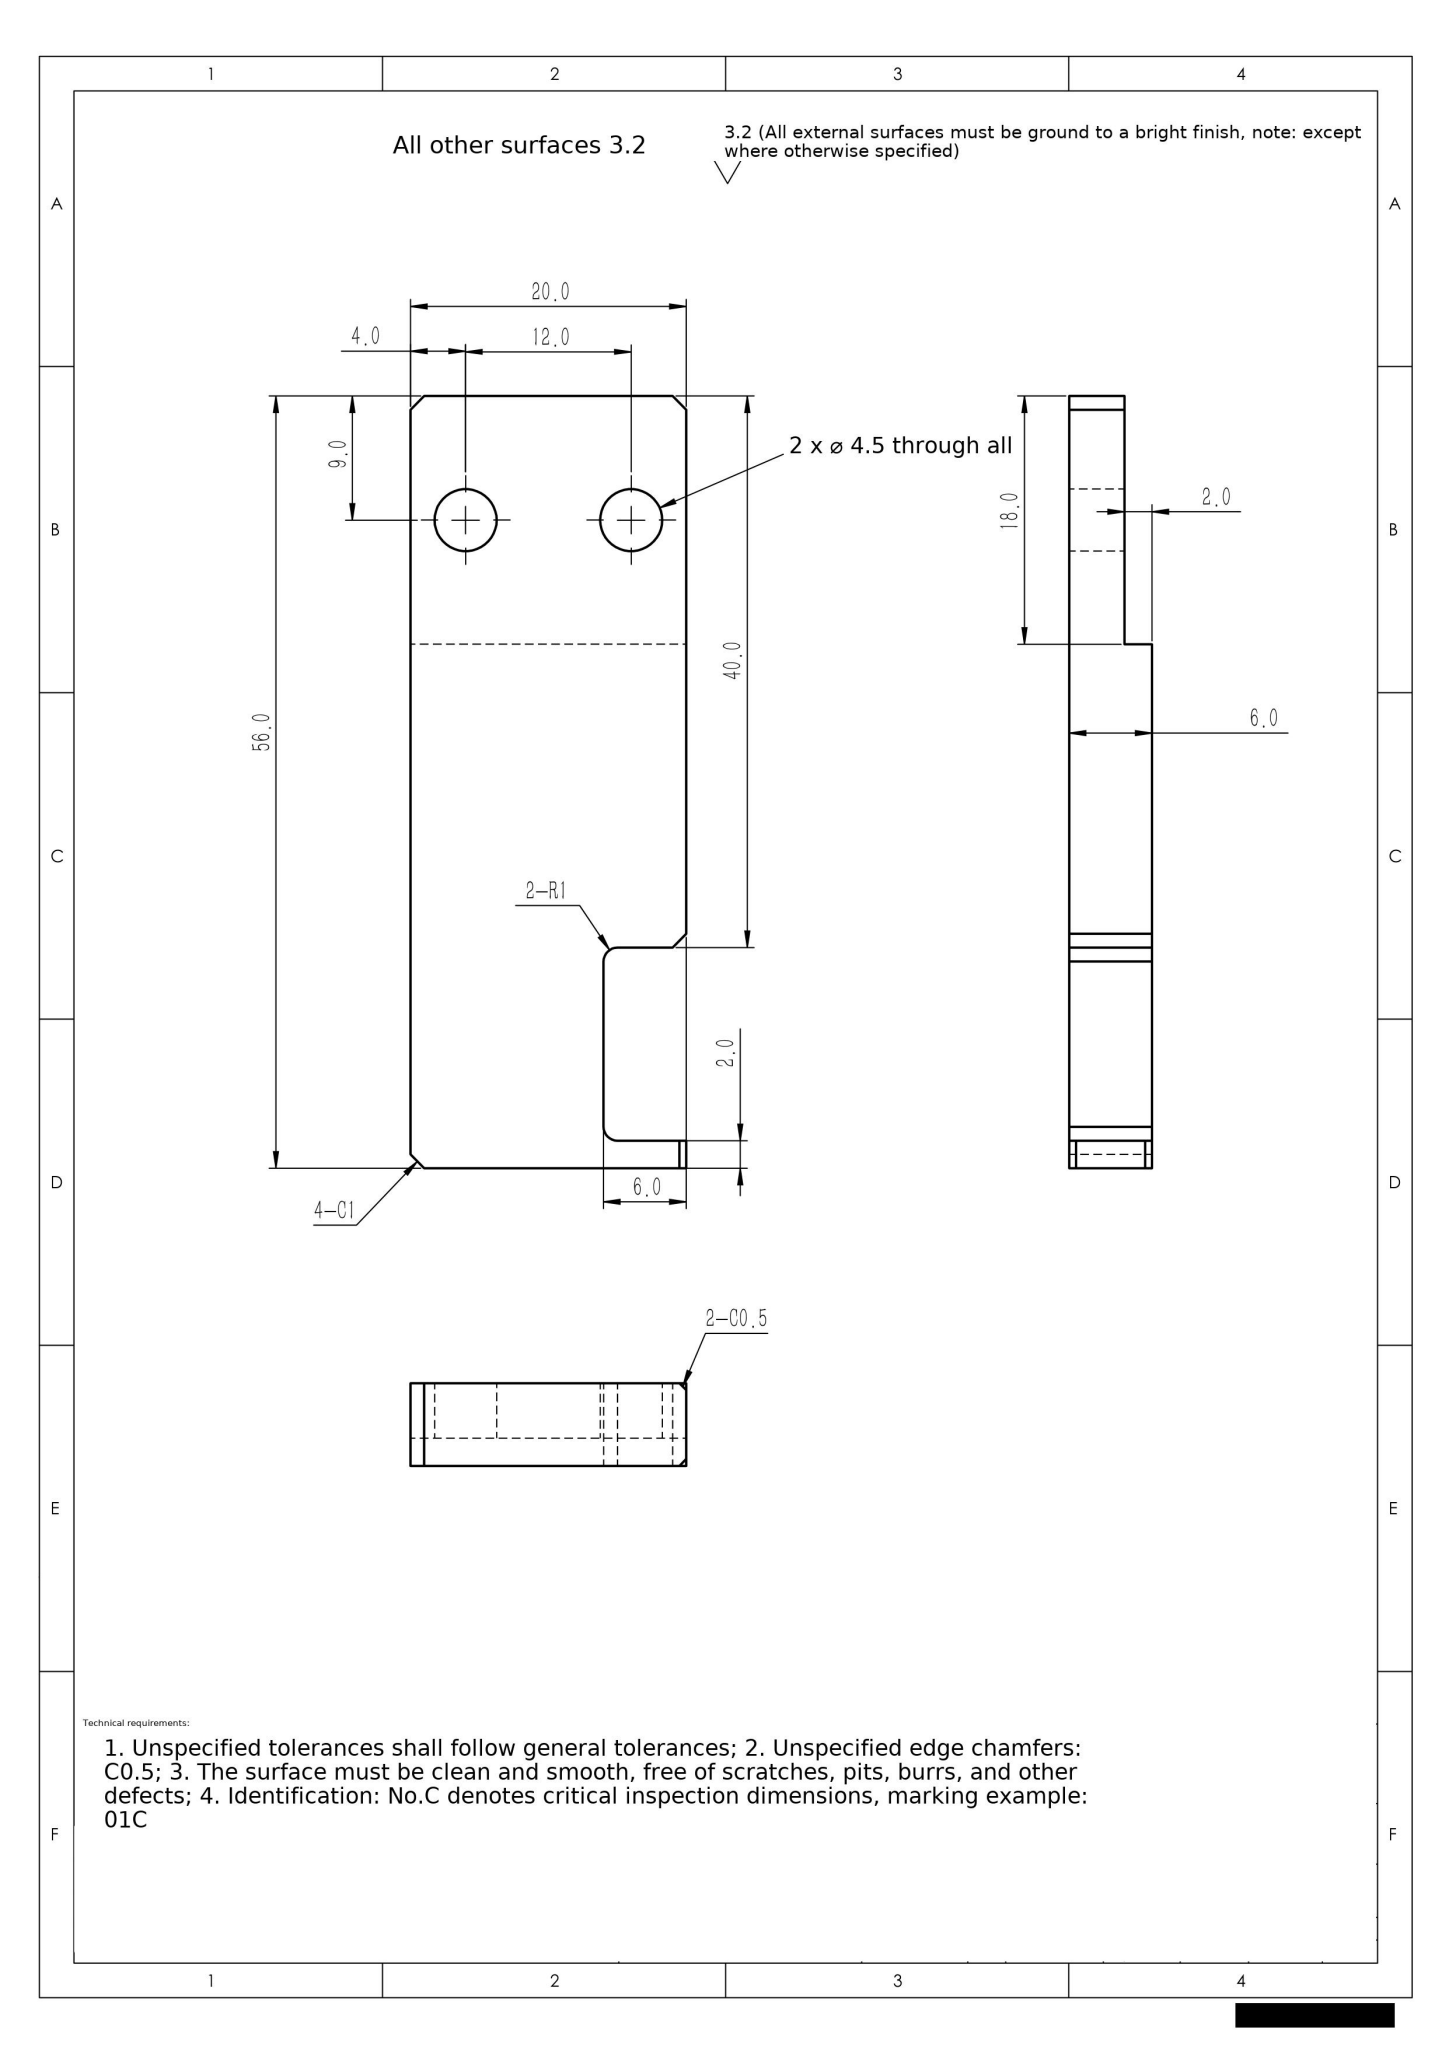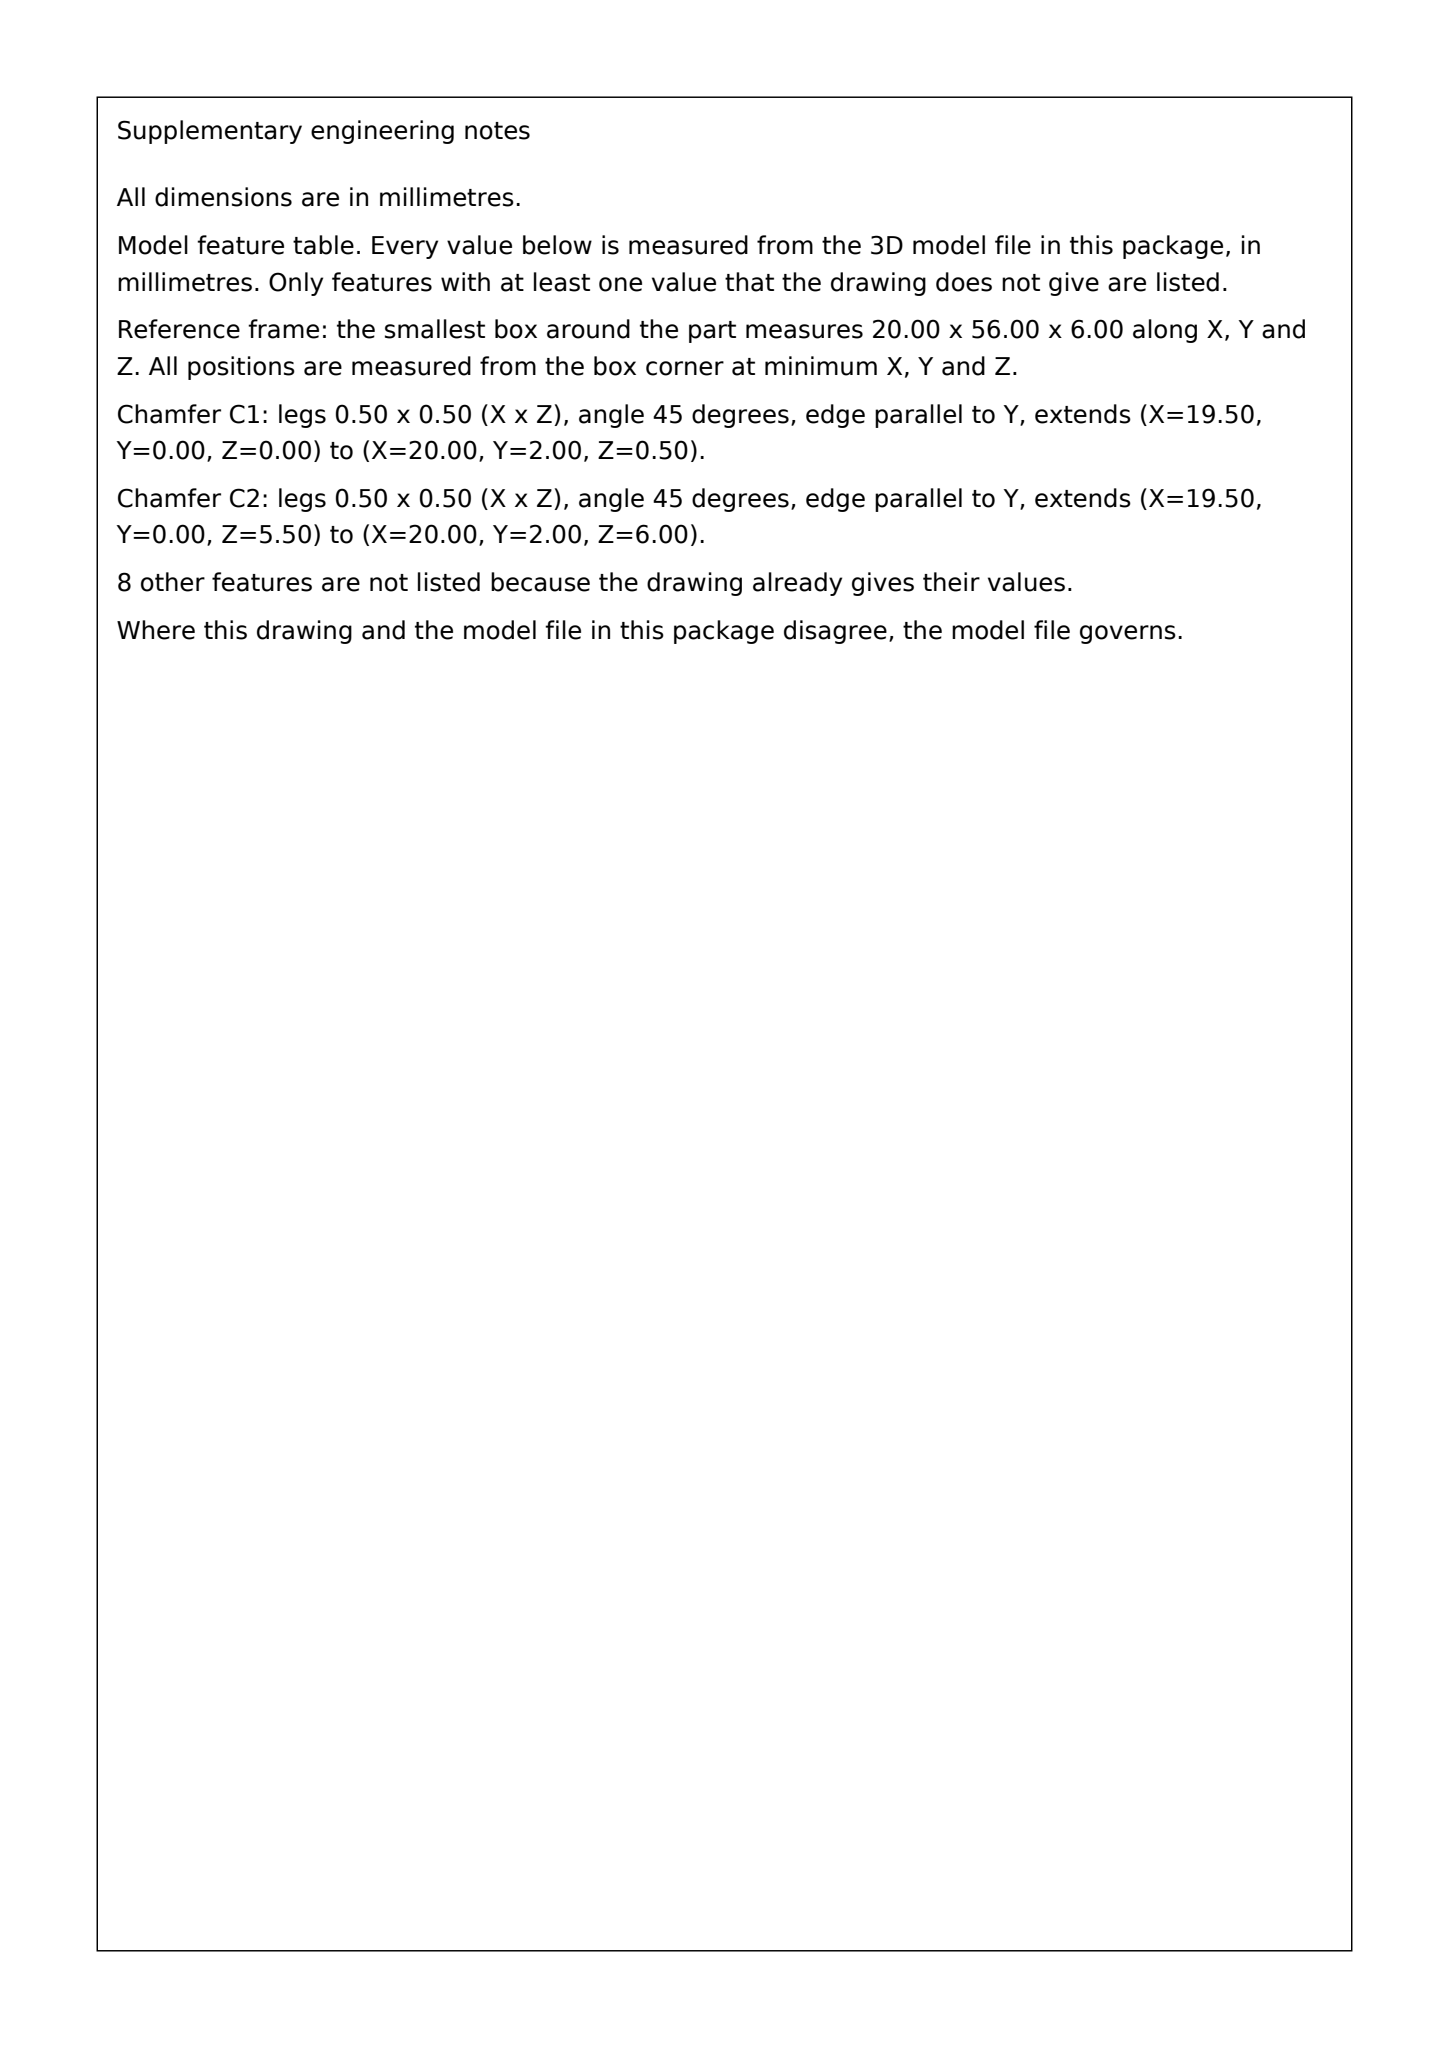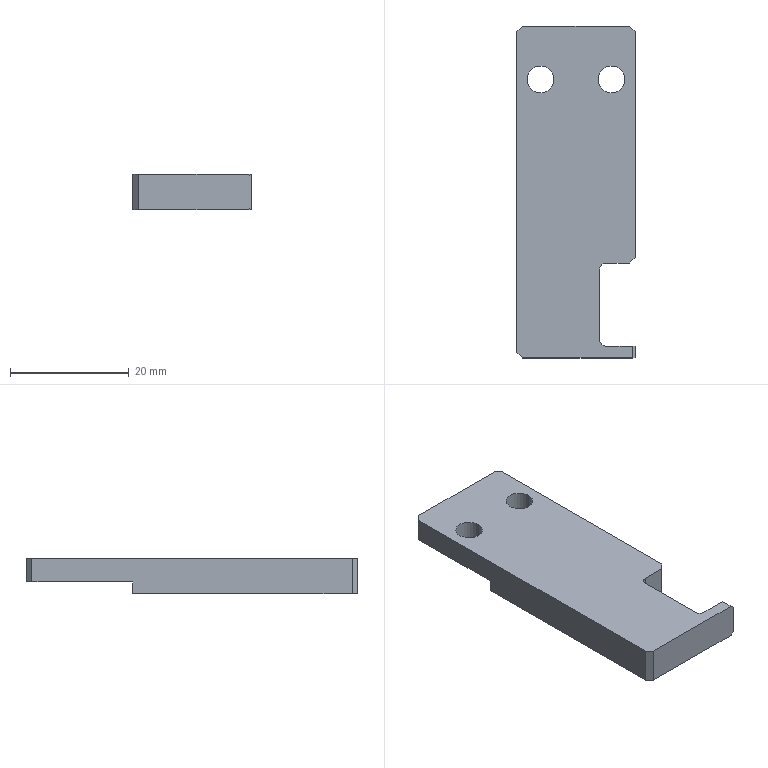Part | SolidWorks | mm | 1 solid | 24 faces | box 20 x 56 x 6 mm | volume 5361 mm3 | plane 18 | cylinder 6 | commonest cylinder face diameters 4.5 x4 2 x2
build123d program:
from build123d import *

# Parameters (mm, degrees)
SKETCH1_W                  = 20
SKETCH1_H                  = 56
BOSS_EXTRUDE1_DEPTH        = 3
F_4_5_4_5_DIAMETER_HOLE2_D = 4.5
SKETCH9_W                  = 6
SKETCH9_H                  = 14
CUT_EXTRUDE1_DEPTH         = 60.766
SKETCH10_W                 = 20
SKETCH10_H                 = 18
CUT_EXTRUDE2_DEPTH         = 2
CHAMFER1_SIZE              = 1
FILLET1_R                  = 1
CHAMFER2_SIZE              = 0.5


with BuildPart() as part:
    # Sketch1 → Boss-Extrude1 (new, symmetric)
    with BuildSketch(Plane.XY):
        with Locations((-10, 28)):
            Rectangle(SKETCH1_W, SKETCH1_H)
    extrude(amount=BOSS_EXTRUDE1_DEPTH, both=True)

    # 4.5 _4.5_ Diameter Hole2 (through all)
    with Locations(Plane(origin=(0, 0, -3), x_dir=(-1, 0, 0), z_dir=(0, 0, -1))):
        with Locations((4, 47), (16, 47)):
            Hole(F_4_5_4_5_DIAMETER_HOLE2_D / 2)

    # Sketch9 → Cut-Extrude1 (cut, through all)
    with BuildSketch(Plane.XY.offset(3)):
        with Locations((-3, 9)):
            Rectangle(SKETCH9_W, SKETCH9_H)
    extrude(amount=-CUT_EXTRUDE1_DEPTH, mode=Mode.SUBTRACT)

    # Sketch10 → Cut-Extrude2 (cut)
    with BuildSketch(Plane(origin=(0, 0, -3), x_dir=(-1, 0, 0), z_dir=(0, 0, -1))):
        with Locations((10, 47)):
            Rectangle(SKETCH10_W, SKETCH10_H)
    extrude(amount=-CUT_EXTRUDE2_DEPTH, mode=Mode.SUBTRACT)

    # Chamfer1
    chamfer1_edges = [part.edges().sort_by_distance(p)[0] for p in [
        (0, 16, 0),
        (-20, 0, 0),
        (-20, 56, 1),
        (0, 56, 1),
    ]]
    chamfer(chamfer1_edges, length=CHAMFER1_SIZE)

    # Fillet1
    fillet1_edges = [part.edges().sort_by_distance(p)[0] for p in [
        (-6, 2, 0),
        (-6, 16, 0),
    ]]
    fillet(fillet1_edges, radius=FILLET1_R)

    # Chamfer2
    chamfer2_edges = [part.edges().sort_by_distance(p)[0] for p in [
        (0, 1, 3),
        (0, 1, -3),
    ]]
    chamfer(chamfer2_edges, length=CHAMFER2_SIZE)


solid = part.part
STEP:
#1=CARTESIAN_POINT('',(-1.75,47.,3.));
#2=VERTEX_POINT('',#1);
#3=CARTESIAN_POINT('',(-6.25,47.,3.));
#4=VERTEX_POINT('',#3);
#5=CARTESIAN_POINT('',(-4.,47.,3.));
#6=DIRECTION('',(0.,0.,-1.));
#7=DIRECTION('',(-1.,0.,0.));
#8=AXIS2_PLACEMENT_3D('',#5,#6,#7);
#9=CIRCLE('',#8,2.25);
#10=EDGE_CURVE('',#2,#4,#9,.T.);
#11=ORIENTED_EDGE('',*,*,#10,.F.);
#12=CARTESIAN_POINT('',(-1.75,47.,-1.));
#13=VERTEX_POINT('',#12);
#14=CARTESIAN_POINT('',(-1.75,47.,-3.));
#15=DIRECTION('',(0.,0.,-1.));
#16=VECTOR('',#15,1000.);
#17=LINE('',#14,#16);
#18=EDGE_CURVE('',#2,#13,#17,.T.);
#19=ORIENTED_EDGE('',*,*,#18,.T.);
#20=CARTESIAN_POINT('',(-6.25,47.,-1.));
#21=VERTEX_POINT('',#20);
#22=CARTESIAN_POINT('',(-4.,47.,-1.));
#23=DIRECTION('',(0.,0.,-1.));
#24=DIRECTION('',(1.,0.,0.));
#25=AXIS2_PLACEMENT_3D('',#22,#23,#24);
#26=CIRCLE('',#25,2.25);
#27=EDGE_CURVE('',#13,#21,#26,.T.);
#28=ORIENTED_EDGE('',*,*,#27,.T.);
#29=CARTESIAN_POINT('',(-6.25,47.,-3.));
#30=DIRECTION('',(0.,0.,-1.));
#31=VECTOR('',#30,1000.);
#32=LINE('',#29,#31);
#33=EDGE_CURVE('',#4,#21,#32,.T.);
#34=ORIENTED_EDGE('',*,*,#33,.F.);
#35=EDGE_LOOP('',(#11,#19,#28,#34));
#36=FACE_OUTER_BOUND('',#35,.T.);
#37=CARTESIAN_POINT('',(-4.,47.,-3.));
#38=DIRECTION('',(0.,0.,-1.));
#39=DIRECTION('',(-1.,0.,0.));
#40=AXIS2_PLACEMENT_3D('',#37,#38,#39);
#41=CYLINDRICAL_SURFACE('',#40,2.25);
#42=ADVANCED_FACE('',(#36),#41,.F.);
#43=CARTESIAN_POINT('',(-13.75,47.,3.));
#44=VERTEX_POINT('',#43);
#45=CARTESIAN_POINT('',(-18.25,47.,3.));
#46=VERTEX_POINT('',#45);
#47=CARTESIAN_POINT('',(-16.,47.,3.));
#48=DIRECTION('',(0.,0.,-1.));
#49=DIRECTION('',(-1.,0.,0.));
#50=AXIS2_PLACEMENT_3D('',#47,#48,#49);
#51=CIRCLE('',#50,2.25);
#52=EDGE_CURVE('',#44,#46,#51,.T.);
#53=ORIENTED_EDGE('',*,*,#52,.F.);
#54=CARTESIAN_POINT('',(-13.75,47.,-1.));
#55=VERTEX_POINT('',#54);
#56=CARTESIAN_POINT('',(-13.75,47.,-3.));
#57=DIRECTION('',(0.,0.,-1.));
#58=VECTOR('',#57,1000.);
#59=LINE('',#56,#58);
#60=EDGE_CURVE('',#44,#55,#59,.T.);
#61=ORIENTED_EDGE('',*,*,#60,.T.);
#62=CARTESIAN_POINT('',(-18.25,47.,-1.));
#63=VERTEX_POINT('',#62);
#64=CARTESIAN_POINT('',(-16.,47.,-1.));
#65=DIRECTION('',(0.,0.,-1.));
#66=DIRECTION('',(1.,0.,0.));
#67=AXIS2_PLACEMENT_3D('',#64,#65,#66);
#68=CIRCLE('',#67,2.25);
#69=EDGE_CURVE('',#55,#63,#68,.T.);
#70=ORIENTED_EDGE('',*,*,#69,.T.);
#71=CARTESIAN_POINT('',(-18.25,47.,-3.));
#72=DIRECTION('',(0.,0.,-1.));
#73=VECTOR('',#72,1000.);
#74=LINE('',#71,#73);
#75=EDGE_CURVE('',#46,#63,#74,.T.);
#76=ORIENTED_EDGE('',*,*,#75,.F.);
#77=EDGE_LOOP('',(#53,#61,#70,#76));
#78=FACE_OUTER_BOUND('',#77,.T.);
#79=CARTESIAN_POINT('',(-16.,47.,-3.));
#80=DIRECTION('',(0.,0.,-1.));
#81=DIRECTION('',(-1.,0.,0.));
#82=AXIS2_PLACEMENT_3D('',#79,#80,#81);
#83=CYLINDRICAL_SURFACE('',#82,2.25);
#84=ADVANCED_FACE('',(#78),#83,.F.);
#85=CARTESIAN_POINT('',(0.,0.,2.5));
#86=VERTEX_POINT('',#85);
#87=CARTESIAN_POINT('',(0.,0.,-2.5));
#88=VERTEX_POINT('',#87);
#89=CARTESIAN_POINT('',(0.,0.,3.));
#90=DIRECTION('',(0.,0.,-1.));
#91=VECTOR('',#90,1000.);
#92=LINE('',#89,#91);
#93=EDGE_CURVE('',#86,#88,#92,.T.);
#94=ORIENTED_EDGE('',*,*,#93,.T.);
#95=CARTESIAN_POINT('',(0.,2.,-2.5));
#96=VERTEX_POINT('',#95);
#97=CARTESIAN_POINT('',(0.,2.,-2.5));
#98=DIRECTION('',(0.,1.,0.));
#99=VECTOR('',#98,1000.);
#100=LINE('',#97,#99);
#101=EDGE_CURVE('',#88,#96,#100,.T.);
#102=ORIENTED_EDGE('',*,*,#101,.T.);
#103=CARTESIAN_POINT('',(0.,2.,2.5));
#104=VERTEX_POINT('',#103);
#105=CARTESIAN_POINT('',(0.,2.,-3.));
#106=DIRECTION('',(0.,0.,1.));
#107=VECTOR('',#106,1000.);
#108=LINE('',#105,#107);
#109=EDGE_CURVE('',#96,#104,#108,.T.);
#110=ORIENTED_EDGE('',*,*,#109,.T.);
#111=CARTESIAN_POINT('',(0.,56.,2.5));
#112=DIRECTION('',(-0.,-1.,0.));
#113=VECTOR('',#112,1000.);
#114=LINE('',#111,#113);
#115=EDGE_CURVE('',#104,#86,#114,.T.);
#116=ORIENTED_EDGE('',*,*,#115,.T.);
#117=EDGE_LOOP('',(#94,#102,#110,#116));
#118=FACE_OUTER_BOUND('',#117,.T.);
#119=CARTESIAN_POINT('',(0.,56.,3.));
#120=DIRECTION('',(-1.,0.,0.));
#121=DIRECTION('',(-0.,-1.,0.));
#122=AXIS2_PLACEMENT_3D('',#119,#120,#121);
#123=PLANE('',#122);
#124=ADVANCED_FACE('',(#118),#123,.F.);
#125=CARTESIAN_POINT('',(0.,17.,3.));
#126=VERTEX_POINT('',#125);
#127=CARTESIAN_POINT('',(0.,55.,3.));
#128=VERTEX_POINT('',#127);
#129=CARTESIAN_POINT('',(0.,56.,3.));
#130=DIRECTION('',(0.,1.,0.));
#131=VECTOR('',#130,1000.);
#132=LINE('',#129,#131);
#133=EDGE_CURVE('',#126,#128,#132,.T.);
#134=ORIENTED_EDGE('',*,*,#133,.F.);
#135=CARTESIAN_POINT('',(0.,17.,-3.));
#136=VERTEX_POINT('',#135);
#137=CARTESIAN_POINT('',(0.,17.,3.));
#138=DIRECTION('',(0.,0.,-1.));
#139=VECTOR('',#138,1000.);
#140=LINE('',#137,#139);
#141=EDGE_CURVE('',#126,#136,#140,.T.);
#142=ORIENTED_EDGE('',*,*,#141,.T.);
#143=CARTESIAN_POINT('',(0.,38.,-3.));
#144=VERTEX_POINT('',#143);
#145=CARTESIAN_POINT('',(0.,56.,-3.));
#146=DIRECTION('',(0.,1.,0.));
#147=VECTOR('',#146,1000.);
#148=LINE('',#145,#147);
#149=EDGE_CURVE('',#136,#144,#148,.T.);
#150=ORIENTED_EDGE('',*,*,#149,.T.);
#151=CARTESIAN_POINT('',(0.,38.,-1.));
#152=VERTEX_POINT('',#151);
#153=CARTESIAN_POINT('',(0.,38.,-1.));
#154=DIRECTION('',(0.,0.,-1.));
#155=VECTOR('',#154,1000.);
#156=LINE('',#153,#155);
#157=EDGE_CURVE('',#152,#144,#156,.T.);
#158=ORIENTED_EDGE('',*,*,#157,.F.);
#159=CARTESIAN_POINT('',(0.,55.,-1.));
#160=VERTEX_POINT('',#159);
#161=CARTESIAN_POINT('',(0.,56.,-1.));
#162=DIRECTION('',(-0.,-1.,0.));
#163=VECTOR('',#162,1000.);
#164=LINE('',#161,#163);
#165=EDGE_CURVE('',#160,#152,#164,.T.);
#166=ORIENTED_EDGE('',*,*,#165,.F.);
#167=CARTESIAN_POINT('',(0.,55.,3.));
#168=DIRECTION('',(0.,0.,1.));
#169=VECTOR('',#168,1000.);
#170=LINE('',#167,#169);
#171=EDGE_CURVE('',#160,#128,#170,.T.);
#172=ORIENTED_EDGE('',*,*,#171,.T.);
#173=EDGE_LOOP('',(#134,#142,#150,#158,#166,#172));
#174=FACE_OUTER_BOUND('',#173,.T.);
#175=CARTESIAN_POINT('',(0.,56.,3.));
#176=DIRECTION('',(-1.,0.,0.));
#177=DIRECTION('',(-0.,-1.,0.));
#178=AXIS2_PLACEMENT_3D('',#175,#176,#177);
#179=PLANE('',#178);
#180=ADVANCED_FACE('',(#174),#179,.F.);
#181=CARTESIAN_POINT('',(-19.,56.,-1.));
#182=VERTEX_POINT('',#181);
#183=CARTESIAN_POINT('',(-1.,56.,-1.));
#184=VERTEX_POINT('',#183);
#185=CARTESIAN_POINT('',(-20.,56.,-1.));
#186=DIRECTION('',(1.,0.,0.));
#187=VECTOR('',#186,1000.);
#188=LINE('',#185,#187);
#189=EDGE_CURVE('',#182,#184,#188,.T.);
#190=ORIENTED_EDGE('',*,*,#189,.F.);
#191=CARTESIAN_POINT('',(-19.,56.,3.));
#192=VERTEX_POINT('',#191);
#193=CARTESIAN_POINT('',(-19.,56.,3.));
#194=DIRECTION('',(0.,0.,1.));
#195=VECTOR('',#194,1000.);
#196=LINE('',#193,#195);
#197=EDGE_CURVE('',#182,#192,#196,.T.);
#198=ORIENTED_EDGE('',*,*,#197,.T.);
#199=CARTESIAN_POINT('',(-1.,56.,3.));
#200=VERTEX_POINT('',#199);
#201=CARTESIAN_POINT('',(0.,56.,3.));
#202=DIRECTION('',(-1.,0.,0.));
#203=VECTOR('',#202,1000.);
#204=LINE('',#201,#203);
#205=EDGE_CURVE('',#200,#192,#204,.T.);
#206=ORIENTED_EDGE('',*,*,#205,.F.);
#207=CARTESIAN_POINT('',(-1.,56.,3.));
#208=DIRECTION('',(0.,0.,-1.));
#209=VECTOR('',#208,1000.);
#210=LINE('',#207,#209);
#211=EDGE_CURVE('',#200,#184,#210,.T.);
#212=ORIENTED_EDGE('',*,*,#211,.T.);
#213=EDGE_LOOP('',(#190,#198,#206,#212));
#214=FACE_OUTER_BOUND('',#213,.T.);
#215=CARTESIAN_POINT('',(0.,56.,3.));
#216=DIRECTION('',(0.,-1.,0.));
#217=DIRECTION('',(0.,0.,-1.));
#218=AXIS2_PLACEMENT_3D('',#215,#216,#217);
#219=PLANE('',#218);
#220=ADVANCED_FACE('',(#214),#219,.F.);
#221=CARTESIAN_POINT('',(-20.,38.,-3.));
#222=VERTEX_POINT('',#221);
#223=CARTESIAN_POINT('',(-20.,1.,-3.));
#224=VERTEX_POINT('',#223);
#225=CARTESIAN_POINT('',(-20.,-0.,-3.));
#226=DIRECTION('',(0.,-1.,0.));
#227=VECTOR('',#226,1000.);
#228=LINE('',#225,#227);
#229=EDGE_CURVE('',#222,#224,#228,.T.);
#230=ORIENTED_EDGE('',*,*,#229,.T.);
#231=CARTESIAN_POINT('',(-20.,1.,3.));
#232=VERTEX_POINT('',#231);
#233=CARTESIAN_POINT('',(-20.,1.,3.));
#234=DIRECTION('',(0.,0.,1.));
#235=VECTOR('',#234,1000.);
#236=LINE('',#233,#235);
#237=EDGE_CURVE('',#224,#232,#236,.T.);
#238=ORIENTED_EDGE('',*,*,#237,.T.);
#239=CARTESIAN_POINT('',(-20.,55.,3.));
#240=VERTEX_POINT('',#239);
#241=CARTESIAN_POINT('',(-20.,-0.,3.));
#242=DIRECTION('',(0.,-1.,0.));
#243=VECTOR('',#242,1000.);
#244=LINE('',#241,#243);
#245=EDGE_CURVE('',#240,#232,#244,.T.);
#246=ORIENTED_EDGE('',*,*,#245,.F.);
#247=CARTESIAN_POINT('',(-20.,55.,-1.));
#248=VERTEX_POINT('',#247);
#249=CARTESIAN_POINT('',(-20.,55.,3.));
#250=DIRECTION('',(0.,0.,-1.));
#251=VECTOR('',#250,1000.);
#252=LINE('',#249,#251);
#253=EDGE_CURVE('',#240,#248,#252,.T.);
#254=ORIENTED_EDGE('',*,*,#253,.T.);
#255=CARTESIAN_POINT('',(-20.,38.,-1.));
#256=VERTEX_POINT('',#255);
#257=CARTESIAN_POINT('',(-20.,56.,-1.));
#258=DIRECTION('',(0.,1.,0.));
#259=VECTOR('',#258,1000.);
#260=LINE('',#257,#259);
#261=EDGE_CURVE('',#256,#248,#260,.T.);
#262=ORIENTED_EDGE('',*,*,#261,.F.);
#263=CARTESIAN_POINT('',(-20.,38.,-1.));
#264=DIRECTION('',(0.,0.,-1.));
#265=VECTOR('',#264,1000.);
#266=LINE('',#263,#265);
#267=EDGE_CURVE('',#256,#222,#266,.T.);
#268=ORIENTED_EDGE('',*,*,#267,.T.);
#269=EDGE_LOOP('',(#230,#238,#246,#254,#262,#268));
#270=FACE_OUTER_BOUND('',#269,.T.);
#271=CARTESIAN_POINT('',(-20.,-0.,3.));
#272=DIRECTION('',(1.,0.,0.));
#273=DIRECTION('',(-0.,1.,0.));
#274=AXIS2_PLACEMENT_3D('',#271,#272,#273);
#275=PLANE('',#274);
#276=ADVANCED_FACE('',(#270),#275,.F.);
#277=CARTESIAN_POINT('',(-19.,-0.,-3.));
#278=VERTEX_POINT('',#277);
#279=CARTESIAN_POINT('',(-0.5,-0.,-3.));
#280=VERTEX_POINT('',#279);
#281=CARTESIAN_POINT('',(0.,0.,-3.));
#282=DIRECTION('',(1.,0.,0.));
#283=VECTOR('',#282,1000.);
#284=LINE('',#281,#283);
#285=EDGE_CURVE('',#278,#280,#284,.T.);
#286=ORIENTED_EDGE('',*,*,#285,.T.);
#287=CARTESIAN_POINT('',(0.,0.,-2.5));
#288=DIRECTION('',(0.7071,0.,0.7071));
#289=VECTOR('',#288,1000.);
#290=LINE('',#287,#289);
#291=EDGE_CURVE('',#280,#88,#290,.T.);
#292=ORIENTED_EDGE('',*,*,#291,.T.);
#293=ORIENTED_EDGE('',*,*,#93,.F.);
#294=CARTESIAN_POINT('',(-0.5,-0.,3.));
#295=VERTEX_POINT('',#294);
#296=CARTESIAN_POINT('',(-0.5,-0.,3.));
#297=DIRECTION('',(-0.7071,-0.,0.7071));
#298=VECTOR('',#297,1000.);
#299=LINE('',#296,#298);
#300=EDGE_CURVE('',#86,#295,#299,.T.);
#301=ORIENTED_EDGE('',*,*,#300,.T.);
#302=CARTESIAN_POINT('',(-19.,-0.,3.));
#303=VERTEX_POINT('',#302);
#304=CARTESIAN_POINT('',(0.,0.,3.));
#305=DIRECTION('',(1.,0.,0.));
#306=VECTOR('',#305,1000.);
#307=LINE('',#304,#306);
#308=EDGE_CURVE('',#303,#295,#307,.T.);
#309=ORIENTED_EDGE('',*,*,#308,.F.);
#310=CARTESIAN_POINT('',(-19.,-0.,3.));
#311=DIRECTION('',(0.,0.,-1.));
#312=VECTOR('',#311,1000.);
#313=LINE('',#310,#312);
#314=EDGE_CURVE('',#303,#278,#313,.T.);
#315=ORIENTED_EDGE('',*,*,#314,.T.);
#316=EDGE_LOOP('',(#286,#292,#293,#301,#309,#315));
#317=FACE_OUTER_BOUND('',#316,.T.);
#318=CARTESIAN_POINT('',(0.,0.,3.));
#319=DIRECTION('',(-0.,1.,0.));
#320=DIRECTION('',(-1.,-0.,0.));
#321=AXIS2_PLACEMENT_3D('',#318,#319,#320);
#322=PLANE('',#321);
#323=ADVANCED_FACE('',(#317),#322,.F.);
#324=CARTESIAN_POINT('',(-4.,47.,3.));
#325=DIRECTION('',(0.,0.,-1.));
#326=DIRECTION('',(-1.,0.,0.));
#327=AXIS2_PLACEMENT_3D('',#324,#325,#326);
#328=CIRCLE('',#327,2.25);
#329=EDGE_CURVE('',#4,#2,#328,.T.);
#330=ORIENTED_EDGE('',*,*,#329,.T.);
#331=ORIENTED_EDGE('',*,*,#10,.T.);
#332=EDGE_LOOP('',(#330,#331));
#333=FACE_BOUND('',#332,.T.);
#334=CARTESIAN_POINT('',(-16.,47.,3.));
#335=DIRECTION('',(0.,0.,-1.));
#336=DIRECTION('',(-1.,0.,0.));
#337=AXIS2_PLACEMENT_3D('',#334,#335,#336);
#338=CIRCLE('',#337,2.25);
#339=EDGE_CURVE('',#46,#44,#338,.T.);
#340=ORIENTED_EDGE('',*,*,#339,.T.);
#341=ORIENTED_EDGE('',*,*,#52,.T.);
#342=EDGE_LOOP('',(#340,#341));
#343=FACE_BOUND('',#342,.T.);
#344=ORIENTED_EDGE('',*,*,#308,.T.);
#345=CARTESIAN_POINT('',(-0.5,2.,3.));
#346=VERTEX_POINT('',#345);
#347=CARTESIAN_POINT('',(-0.5,0.,3.));
#348=DIRECTION('',(0.,1.,0.));
#349=VECTOR('',#348,1000.);
#350=LINE('',#347,#349);
#351=EDGE_CURVE('',#295,#346,#350,.T.);
#352=ORIENTED_EDGE('',*,*,#351,.T.);
#353=CARTESIAN_POINT('',(-5.,2.,3.));
#354=VERTEX_POINT('',#353);
#355=CARTESIAN_POINT('',(0.,2.,3.));
#356=DIRECTION('',(1.,0.,0.));
#357=VECTOR('',#356,1000.);
#358=LINE('',#355,#357);
#359=EDGE_CURVE('',#354,#346,#358,.T.);
#360=ORIENTED_EDGE('',*,*,#359,.F.);
#361=CARTESIAN_POINT('',(-6.,3.,3.));
#362=VERTEX_POINT('',#361);
#363=CARTESIAN_POINT('',(-5.,3.,3.));
#364=DIRECTION('',(0.,0.,-1.));
#365=DIRECTION('',(-1.,0.,0.));
#366=AXIS2_PLACEMENT_3D('',#363,#364,#365);
#367=CIRCLE('',#366,1.);
#368=EDGE_CURVE('',#354,#362,#367,.T.);
#369=ORIENTED_EDGE('',*,*,#368,.T.);
#370=CARTESIAN_POINT('',(-6.,15.,3.));
#371=VERTEX_POINT('',#370);
#372=CARTESIAN_POINT('',(-6.,2.,3.));
#373=DIRECTION('',(0.,-1.,0.));
#374=VECTOR('',#373,1000.);
#375=LINE('',#372,#374);
#376=EDGE_CURVE('',#371,#362,#375,.T.);
#377=ORIENTED_EDGE('',*,*,#376,.F.);
#378=CARTESIAN_POINT('',(-5.,16.,3.));
#379=VERTEX_POINT('',#378);
#380=CARTESIAN_POINT('',(-5.,15.,3.));
#381=DIRECTION('',(0.,0.,-1.));
#382=DIRECTION('',(-1.,0.,0.));
#383=AXIS2_PLACEMENT_3D('',#380,#381,#382);
#384=CIRCLE('',#383,1.);
#385=EDGE_CURVE('',#371,#379,#384,.T.);
#386=ORIENTED_EDGE('',*,*,#385,.T.);
#387=CARTESIAN_POINT('',(-1.,16.,3.));
#388=VERTEX_POINT('',#387);
#389=CARTESIAN_POINT('',(0.,16.,3.));
#390=DIRECTION('',(-1.,0.,0.));
#391=VECTOR('',#390,1000.);
#392=LINE('',#389,#391);
#393=EDGE_CURVE('',#388,#379,#392,.T.);
#394=ORIENTED_EDGE('',*,*,#393,.F.);
#395=CARTESIAN_POINT('',(-1.,16.,3.));
#396=DIRECTION('',(0.7071,0.7071,0.));
#397=VECTOR('',#396,1000.);
#398=LINE('',#395,#397);
#399=EDGE_CURVE('',#388,#126,#398,.T.);
#400=ORIENTED_EDGE('',*,*,#399,.T.);
#401=ORIENTED_EDGE('',*,*,#133,.T.);
#402=CARTESIAN_POINT('',(-1.,56.,3.));
#403=DIRECTION('',(-0.7071,0.7071,0.));
#404=VECTOR('',#403,1000.);
#405=LINE('',#402,#404);
#406=EDGE_CURVE('',#128,#200,#405,.T.);
#407=ORIENTED_EDGE('',*,*,#406,.T.);
#408=ORIENTED_EDGE('',*,*,#205,.T.);
#409=CARTESIAN_POINT('',(-20.,55.,3.));
#410=DIRECTION('',(-0.7071,-0.7071,0.));
#411=VECTOR('',#410,1000.);
#412=LINE('',#409,#411);
#413=EDGE_CURVE('',#192,#240,#412,.T.);
#414=ORIENTED_EDGE('',*,*,#413,.T.);
#415=ORIENTED_EDGE('',*,*,#245,.T.);
#416=CARTESIAN_POINT('',(-19.,-0.,3.));
#417=DIRECTION('',(0.7071,-0.7071,0.));
#418=VECTOR('',#417,1000.);
#419=LINE('',#416,#418);
#420=EDGE_CURVE('',#232,#303,#419,.T.);
#421=ORIENTED_EDGE('',*,*,#420,.T.);
#422=EDGE_LOOP('',(#344,#352,#360,#369,#377,#386,#394,#400,#401,#407,#408,#414,#415,#421));
#423=FACE_OUTER_BOUND('',#422,.T.);
#424=CARTESIAN_POINT('',(0.,0.,3.));
#425=DIRECTION('',(0.,0.,-1.));
#426=DIRECTION('',(-1.,0.,0.));
#427=AXIS2_PLACEMENT_3D('',#424,#425,#426);
#428=PLANE('',#427);
#429=ADVANCED_FACE('',(#333,#343,#423),#428,.F.);
#430=CARTESIAN_POINT('',(-5.,2.,-3.));
#431=VERTEX_POINT('',#430);
#432=CARTESIAN_POINT('',(-0.5,2.,-3.));
#433=VERTEX_POINT('',#432);
#434=CARTESIAN_POINT('',(0.,2.,-3.));
#435=DIRECTION('',(1.,0.,0.));
#436=VECTOR('',#435,1000.);
#437=LINE('',#434,#436);
#438=EDGE_CURVE('',#431,#433,#437,.T.);
#439=ORIENTED_EDGE('',*,*,#438,.T.);
#440=CARTESIAN_POINT('',(-0.5,0.,-3.));
#441=DIRECTION('',(-0.,-1.,0.));
#442=VECTOR('',#441,1000.);
#443=LINE('',#440,#442);
#444=EDGE_CURVE('',#433,#280,#443,.T.);
#445=ORIENTED_EDGE('',*,*,#444,.T.);
#446=ORIENTED_EDGE('',*,*,#285,.F.);
#447=CARTESIAN_POINT('',(-9.5,-9.5,-3.));
#448=DIRECTION('',(-0.7071,0.7071,0.));
#449=VECTOR('',#448,1000.);
#450=LINE('',#447,#449);
#451=EDGE_CURVE('',#278,#224,#450,.T.);
#452=ORIENTED_EDGE('',*,*,#451,.T.);
#453=ORIENTED_EDGE('',*,*,#229,.F.);
#454=CARTESIAN_POINT('',(-20.,38.,-3.));
#455=DIRECTION('',(-1.,0.,0.));
#456=VECTOR('',#455,1000.);
#457=LINE('',#454,#456);
#458=EDGE_CURVE('',#144,#222,#457,.T.);
#459=ORIENTED_EDGE('',*,*,#458,.F.);
#460=ORIENTED_EDGE('',*,*,#149,.F.);
#461=CARTESIAN_POINT('',(-1.,16.,-3.));
#462=VERTEX_POINT('',#461);
#463=CARTESIAN_POINT('',(-8.5,8.5,-3.));
#464=DIRECTION('',(-0.7071,-0.7071,0.));
#465=VECTOR('',#464,1000.);
#466=LINE('',#463,#465);
#467=EDGE_CURVE('',#136,#462,#466,.T.);
#468=ORIENTED_EDGE('',*,*,#467,.T.);
#469=CARTESIAN_POINT('',(-5.,16.,-3.));
#470=VERTEX_POINT('',#469);
#471=CARTESIAN_POINT('',(0.,16.,-3.));
#472=DIRECTION('',(-1.,0.,0.));
#473=VECTOR('',#472,1000.);
#474=LINE('',#471,#473);
#475=EDGE_CURVE('',#462,#470,#474,.T.);
#476=ORIENTED_EDGE('',*,*,#475,.T.);
#477=CARTESIAN_POINT('',(-6.,15.,-3.));
#478=VERTEX_POINT('',#477);
#479=CARTESIAN_POINT('',(-5.,15.,-3.));
#480=DIRECTION('',(0.,0.,1.));
#481=DIRECTION('',(-1.,0.,0.));
#482=AXIS2_PLACEMENT_3D('',#479,#480,#481);
#483=CIRCLE('',#482,1.);
#484=EDGE_CURVE('',#470,#478,#483,.T.);
#485=ORIENTED_EDGE('',*,*,#484,.T.);
#486=CARTESIAN_POINT('',(-6.,3.,-3.));
#487=VERTEX_POINT('',#486);
#488=CARTESIAN_POINT('',(-6.,2.,-3.));
#489=DIRECTION('',(0.,-1.,0.));
#490=VECTOR('',#489,1000.);
#491=LINE('',#488,#490);
#492=EDGE_CURVE('',#478,#487,#491,.T.);
#493=ORIENTED_EDGE('',*,*,#492,.T.);
#494=CARTESIAN_POINT('',(-5.,3.,-3.));
#495=DIRECTION('',(0.,0.,1.));
#496=DIRECTION('',(-1.,0.,0.));
#497=AXIS2_PLACEMENT_3D('',#494,#495,#496);
#498=CIRCLE('',#497,1.);
#499=EDGE_CURVE('',#487,#431,#498,.T.);
#500=ORIENTED_EDGE('',*,*,#499,.T.);
#501=EDGE_LOOP('',(#439,#445,#446,#452,#453,#459,#460,#468,#476,#485,#493,#500));
#502=FACE_OUTER_BOUND('',#501,.T.);
#503=CARTESIAN_POINT('',(0.,0.,-3.));
#504=DIRECTION('',(0.,0.,-1.));
#505=DIRECTION('',(-1.,0.,0.));
#506=AXIS2_PLACEMENT_3D('',#503,#504,#505);
#507=PLANE('',#506);
#508=ADVANCED_FACE('',(#502),#507,.T.);
#509=ORIENTED_EDGE('',*,*,#60,.F.);
#510=ORIENTED_EDGE('',*,*,#339,.F.);
#511=ORIENTED_EDGE('',*,*,#75,.T.);
#512=CARTESIAN_POINT('',(-16.,47.,-1.));
#513=DIRECTION('',(0.,0.,-1.));
#514=DIRECTION('',(1.,0.,0.));
#515=AXIS2_PLACEMENT_3D('',#512,#513,#514);
#516=CIRCLE('',#515,2.25);
#517=EDGE_CURVE('',#63,#55,#516,.T.);
#518=ORIENTED_EDGE('',*,*,#517,.T.);
#519=EDGE_LOOP('',(#509,#510,#511,#518));
#520=FACE_OUTER_BOUND('',#519,.T.);
#521=CARTESIAN_POINT('',(-16.,47.,-3.));
#522=DIRECTION('',(0.,0.,-1.));
#523=DIRECTION('',(-1.,0.,0.));
#524=AXIS2_PLACEMENT_3D('',#521,#522,#523);
#525=CYLINDRICAL_SURFACE('',#524,2.25);
#526=ADVANCED_FACE('',(#520),#525,.F.);
#527=ORIENTED_EDGE('',*,*,#18,.F.);
#528=ORIENTED_EDGE('',*,*,#329,.F.);
#529=ORIENTED_EDGE('',*,*,#33,.T.);
#530=CARTESIAN_POINT('',(-4.,47.,-1.));
#531=DIRECTION('',(0.,0.,-1.));
#532=DIRECTION('',(1.,0.,0.));
#533=AXIS2_PLACEMENT_3D('',#530,#531,#532);
#534=CIRCLE('',#533,2.25);
#535=EDGE_CURVE('',#21,#13,#534,.T.);
#536=ORIENTED_EDGE('',*,*,#535,.T.);
#537=EDGE_LOOP('',(#527,#528,#529,#536));
#538=FACE_OUTER_BOUND('',#537,.T.);
#539=CARTESIAN_POINT('',(-4.,47.,-3.));
#540=DIRECTION('',(0.,0.,-1.));
#541=DIRECTION('',(-1.,0.,0.));
#542=AXIS2_PLACEMENT_3D('',#539,#540,#541);
#543=CYLINDRICAL_SURFACE('',#542,2.25);
#544=ADVANCED_FACE('',(#538),#543,.F.);
#545=ORIENTED_EDGE('',*,*,#109,.F.);
#546=CARTESIAN_POINT('',(0.,2.,-2.5));
#547=DIRECTION('',(-0.7071,-0.,-0.7071));
#548=VECTOR('',#547,1000.);
#549=LINE('',#546,#548);
#550=EDGE_CURVE('',#96,#433,#549,.T.);
#551=ORIENTED_EDGE('',*,*,#550,.T.);
#552=ORIENTED_EDGE('',*,*,#438,.F.);
#553=CARTESIAN_POINT('',(-5.,2.,3.));
#554=DIRECTION('',(0.,0.,1.));
#555=VECTOR('',#554,1000.);
#556=LINE('',#553,#555);
#557=EDGE_CURVE('',#431,#354,#556,.T.);
#558=ORIENTED_EDGE('',*,*,#557,.T.);
#559=ORIENTED_EDGE('',*,*,#359,.T.);
#560=CARTESIAN_POINT('',(-0.5,2.,3.));
#561=DIRECTION('',(0.7071,0.,-0.7071));
#562=VECTOR('',#561,1000.);
#563=LINE('',#560,#562);
#564=EDGE_CURVE('',#346,#104,#563,.T.);
#565=ORIENTED_EDGE('',*,*,#564,.T.);
#566=EDGE_LOOP('',(#545,#551,#552,#558,#559,#565));
#567=FACE_OUTER_BOUND('',#566,.T.);
#568=CARTESIAN_POINT('',(0.,2.,-3.));
#569=DIRECTION('',(0.,-1.,0.));
#570=DIRECTION('',(1.,0.,0.));
#571=AXIS2_PLACEMENT_3D('',#568,#569,#570);
#572=PLANE('',#571);
#573=ADVANCED_FACE('',(#567),#572,.F.);
#574=ORIENTED_EDGE('',*,*,#376,.T.);
#575=CARTESIAN_POINT('',(-6.,3.,-3.));
#576=DIRECTION('',(0.,0.,-1.));
#577=VECTOR('',#576,1000.);
#578=LINE('',#575,#577);
#579=EDGE_CURVE('',#362,#487,#578,.T.);
#580=ORIENTED_EDGE('',*,*,#579,.T.);
#581=ORIENTED_EDGE('',*,*,#492,.F.);
#582=CARTESIAN_POINT('',(-6.,15.,3.));
#583=DIRECTION('',(0.,0.,1.));
#584=VECTOR('',#583,1000.);
#585=LINE('',#582,#584);
#586=EDGE_CURVE('',#478,#371,#585,.T.);
#587=ORIENTED_EDGE('',*,*,#586,.T.);
#588=EDGE_LOOP('',(#574,#580,#581,#587));
#589=FACE_OUTER_BOUND('',#588,.T.);
#590=CARTESIAN_POINT('',(-6.,2.,-3.));
#591=DIRECTION('',(-1.,0.,0.));
#592=DIRECTION('',(0.,0.,1.));
#593=AXIS2_PLACEMENT_3D('',#590,#591,#592);
#594=PLANE('',#593);
#595=ADVANCED_FACE('',(#589),#594,.F.);
#596=ORIENTED_EDGE('',*,*,#393,.T.);
#597=CARTESIAN_POINT('',(-5.,16.,-3.));
#598=DIRECTION('',(0.,0.,-1.));
#599=VECTOR('',#598,1000.);
#600=LINE('',#597,#599);
#601=EDGE_CURVE('',#379,#470,#600,.T.);
#602=ORIENTED_EDGE('',*,*,#601,.T.);
#603=ORIENTED_EDGE('',*,*,#475,.F.);
#604=CARTESIAN_POINT('',(-1.,16.,-3.));
#605=DIRECTION('',(0.,0.,1.));
#606=VECTOR('',#605,1000.);
#607=LINE('',#604,#606);
#608=EDGE_CURVE('',#462,#388,#607,.T.);
#609=ORIENTED_EDGE('',*,*,#608,.T.);
#610=EDGE_LOOP('',(#596,#602,#603,#609));
#611=FACE_OUTER_BOUND('',#610,.T.);
#612=CARTESIAN_POINT('',(0.,16.,-3.));
#613=DIRECTION('',(0.,1.,0.));
#614=DIRECTION('',(0.,0.,1.));
#615=AXIS2_PLACEMENT_3D('',#612,#613,#614);
#616=PLANE('',#615);
#617=ADVANCED_FACE('',(#611),#616,.F.);
#618=ORIENTED_EDGE('',*,*,#535,.F.);
#619=ORIENTED_EDGE('',*,*,#27,.F.);
#620=EDGE_LOOP('',(#618,#619));
#621=FACE_BOUND('',#620,.T.);
#622=ORIENTED_EDGE('',*,*,#261,.T.);
#623=CARTESIAN_POINT('',(-20.,55.,-1.));
#624=DIRECTION('',(0.7071,0.7071,0.));
#625=VECTOR('',#624,1000.);
#626=LINE('',#623,#625);
#627=EDGE_CURVE('',#248,#182,#626,.T.);
#628=ORIENTED_EDGE('',*,*,#627,.T.);
#629=ORIENTED_EDGE('',*,*,#189,.T.);
#630=CARTESIAN_POINT('',(-1.,56.,-1.));
#631=DIRECTION('',(0.7071,-0.7071,0.));
#632=VECTOR('',#631,1000.);
#633=LINE('',#630,#632);
#634=EDGE_CURVE('',#184,#160,#633,.T.);
#635=ORIENTED_EDGE('',*,*,#634,.T.);
#636=ORIENTED_EDGE('',*,*,#165,.T.);
#637=CARTESIAN_POINT('',(-20.,38.,-1.));
#638=DIRECTION('',(-1.,0.,0.));
#639=VECTOR('',#638,1000.);
#640=LINE('',#637,#639);
#641=EDGE_CURVE('',#152,#256,#640,.T.);
#642=ORIENTED_EDGE('',*,*,#641,.T.);
#643=EDGE_LOOP('',(#622,#628,#629,#635,#636,#642));
#644=FACE_OUTER_BOUND('',#643,.T.);
#645=ORIENTED_EDGE('',*,*,#517,.F.);
#646=ORIENTED_EDGE('',*,*,#69,.F.);
#647=EDGE_LOOP('',(#645,#646));
#648=FACE_BOUND('',#647,.T.);
#649=CARTESIAN_POINT('',(0.,0.,-1.));
#650=DIRECTION('',(0.,0.,1.));
#651=DIRECTION('',(1.,0.,0.));
#652=AXIS2_PLACEMENT_3D('',#649,#650,#651);
#653=PLANE('',#652);
#654=ADVANCED_FACE('',(#621,#644,#648),#653,.F.);
#655=ORIENTED_EDGE('',*,*,#458,.T.);
#656=ORIENTED_EDGE('',*,*,#267,.F.);
#657=ORIENTED_EDGE('',*,*,#641,.F.);
#658=ORIENTED_EDGE('',*,*,#157,.T.);
#659=EDGE_LOOP('',(#655,#656,#657,#658));
#660=FACE_OUTER_BOUND('',#659,.T.);
#661=CARTESIAN_POINT('',(-20.,38.,-1.));
#662=DIRECTION('',(0.,-1.,0.));
#663=DIRECTION('',(0.,0.,-1.));
#664=AXIS2_PLACEMENT_3D('',#661,#662,#663);
#665=PLANE('',#664);
#666=ADVANCED_FACE('',(#660),#665,.F.);
#667=ORIENTED_EDGE('',*,*,#467,.F.);
#668=ORIENTED_EDGE('',*,*,#141,.F.);
#669=ORIENTED_EDGE('',*,*,#399,.F.);
#670=ORIENTED_EDGE('',*,*,#608,.F.);
#671=EDGE_LOOP('',(#667,#668,#669,#670));
#672=FACE_OUTER_BOUND('',#671,.T.);
#673=CARTESIAN_POINT('',(-1.,16.,-3.));
#674=DIRECTION('',(-0.7071,0.7071,0.));
#675=DIRECTION('',(0.,0.,1.));
#676=AXIS2_PLACEMENT_3D('',#673,#674,#675);
#677=PLANE('',#676);
#678=ADVANCED_FACE('',(#672),#677,.F.);
#679=ORIENTED_EDGE('',*,*,#420,.F.);
#680=ORIENTED_EDGE('',*,*,#237,.F.);
#681=ORIENTED_EDGE('',*,*,#451,.F.);
#682=ORIENTED_EDGE('',*,*,#314,.F.);
#683=EDGE_LOOP('',(#679,#680,#681,#682));
#684=FACE_OUTER_BOUND('',#683,.T.);
#685=CARTESIAN_POINT('',(-19.,-0.,3.));
#686=DIRECTION('',(0.7071,0.7071,0.));
#687=DIRECTION('',(0.,0.,-1.));
#688=AXIS2_PLACEMENT_3D('',#685,#686,#687);
#689=PLANE('',#688);
#690=ADVANCED_FACE('',(#684),#689,.F.);
#691=ORIENTED_EDGE('',*,*,#413,.F.);
#692=ORIENTED_EDGE('',*,*,#197,.F.);
#693=ORIENTED_EDGE('',*,*,#627,.F.);
#694=ORIENTED_EDGE('',*,*,#253,.F.);
#695=EDGE_LOOP('',(#691,#692,#693,#694));
#696=FACE_OUTER_BOUND('',#695,.T.);
#697=CARTESIAN_POINT('',(-20.,55.,3.));
#698=DIRECTION('',(0.7071,-0.7071,0.));
#699=DIRECTION('',(0.,0.,-1.));
#700=AXIS2_PLACEMENT_3D('',#697,#698,#699);
#701=PLANE('',#700);
#702=ADVANCED_FACE('',(#696),#701,.F.);
#703=ORIENTED_EDGE('',*,*,#406,.F.);
#704=ORIENTED_EDGE('',*,*,#171,.F.);
#705=ORIENTED_EDGE('',*,*,#634,.F.);
#706=ORIENTED_EDGE('',*,*,#211,.F.);
#707=EDGE_LOOP('',(#703,#704,#705,#706));
#708=FACE_OUTER_BOUND('',#707,.T.);
#709=CARTESIAN_POINT('',(-1.,56.,3.));
#710=DIRECTION('',(-0.7071,-0.7071,0.));
#711=DIRECTION('',(0.,0.,-1.));
#712=AXIS2_PLACEMENT_3D('',#709,#710,#711);
#713=PLANE('',#712);
#714=ADVANCED_FACE('',(#708),#713,.F.);
#715=ORIENTED_EDGE('',*,*,#499,.F.);
#716=ORIENTED_EDGE('',*,*,#579,.F.);
#717=ORIENTED_EDGE('',*,*,#368,.F.);
#718=ORIENTED_EDGE('',*,*,#557,.F.);
#719=EDGE_LOOP('',(#715,#716,#717,#718));
#720=FACE_OUTER_BOUND('',#719,.T.);
#721=CARTESIAN_POINT('',(-5.,3.,-3.));
#722=DIRECTION('',(0.,0.,-1.));
#723=DIRECTION('',(-1.,0.,0.));
#724=AXIS2_PLACEMENT_3D('',#721,#722,#723);
#725=CYLINDRICAL_SURFACE('',#724,1.);
#726=ADVANCED_FACE('',(#720),#725,.F.);
#727=ORIENTED_EDGE('',*,*,#484,.F.);
#728=ORIENTED_EDGE('',*,*,#601,.F.);
#729=ORIENTED_EDGE('',*,*,#385,.F.);
#730=ORIENTED_EDGE('',*,*,#586,.F.);
#731=EDGE_LOOP('',(#727,#728,#729,#730));
#732=FACE_OUTER_BOUND('',#731,.T.);
#733=CARTESIAN_POINT('',(-5.,15.,-3.));
#734=DIRECTION('',(0.,0.,-1.));
#735=DIRECTION('',(-1.,0.,0.));
#736=AXIS2_PLACEMENT_3D('',#733,#734,#735);
#737=CYLINDRICAL_SURFACE('',#736,1.);
#738=ADVANCED_FACE('',(#732),#737,.F.);
#739=ORIENTED_EDGE('',*,*,#291,.F.);
#740=ORIENTED_EDGE('',*,*,#444,.F.);
#741=ORIENTED_EDGE('',*,*,#550,.F.);
#742=ORIENTED_EDGE('',*,*,#101,.F.);
#743=EDGE_LOOP('',(#739,#740,#741,#742));
#744=FACE_OUTER_BOUND('',#743,.T.);
#745=CARTESIAN_POINT('',(0.,56.,-2.5));
#746=DIRECTION('',(0.7071,-0.,-0.7071));
#747=DIRECTION('',(-0.,-1.,0.));
#748=AXIS2_PLACEMENT_3D('',#745,#746,#747);
#749=PLANE('',#748);
#750=ADVANCED_FACE('',(#744),#749,.T.);
#751=ORIENTED_EDGE('',*,*,#300,.F.);
#752=ORIENTED_EDGE('',*,*,#115,.F.);
#753=ORIENTED_EDGE('',*,*,#564,.F.);
#754=ORIENTED_EDGE('',*,*,#351,.F.);
#755=EDGE_LOOP('',(#751,#752,#753,#754));
#756=FACE_OUTER_BOUND('',#755,.T.);
#757=CARTESIAN_POINT('',(-0.5,0.,3.));
#758=DIRECTION('',(-0.7071,0.,-0.7071));
#759=DIRECTION('',(0.,1.,0.));
#760=AXIS2_PLACEMENT_3D('',#757,#758,#759);
#761=PLANE('',#760);
#762=ADVANCED_FACE('',(#756),#761,.F.);
#763=CLOSED_SHELL('',(#42,#84,#124,#180,#220,#276,#323,#429,#508,#526,#544,#573,#595,#617,#654,#666,#678,#690,#702,#714,#726,#738,#750,#762));
#764=MANIFOLD_SOLID_BREP('',#763);
#765=CARTESIAN_POINT('',(0.,0.,0.));
#766=DIRECTION('',(0.,0.,1.));
#767=DIRECTION('',(1.,0.,0.));
#768=AXIS2_PLACEMENT_3D('',#765,#766,#767);
#769=(LENGTH_UNIT()NAMED_UNIT(*)SI_UNIT(.MILLI.,.METRE.));
#770=UNCERTAINTY_MEASURE_WITH_UNIT(LENGTH_MEASURE(0.00001),#769,'','');
#771=(NAMED_UNIT(*)PLANE_ANGLE_UNIT()SI_UNIT($,.RADIAN.));
#772=(NAMED_UNIT(*)SI_UNIT($,.STERADIAN.)SOLID_ANGLE_UNIT());
#773=(GEOMETRIC_REPRESENTATION_CONTEXT(3)GLOBAL_UNCERTAINTY_ASSIGNED_CONTEXT((#770))GLOBAL_UNIT_ASSIGNED_CONTEXT((#769,#771,#772))REPRESENTATION_CONTEXT('',''));
#774=ADVANCED_BREP_SHAPE_REPRESENTATION('',(#764,#768),#773);